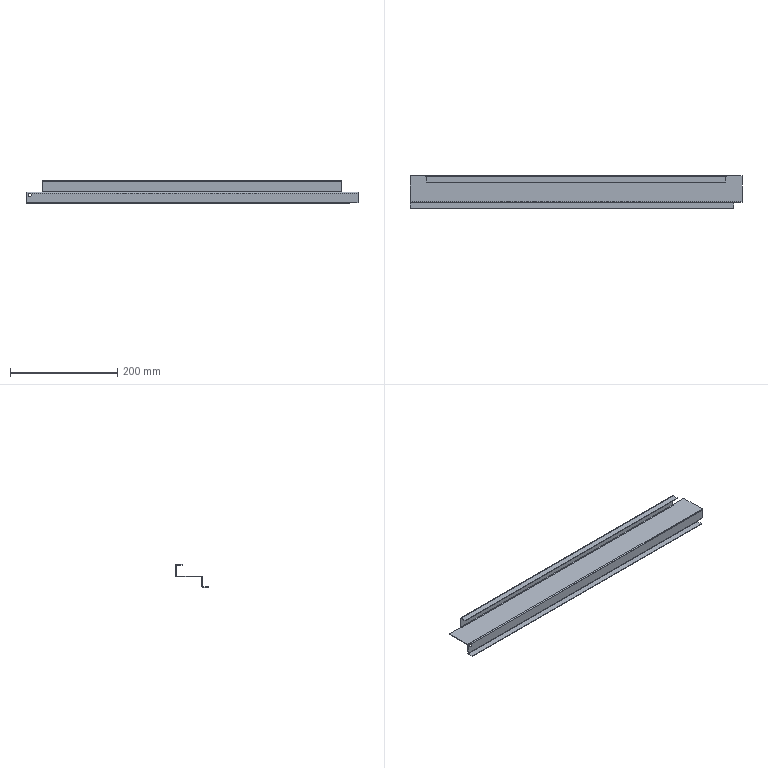Component | SolidWorks | CCQ-1.1-11UpperBeam1-1 | 1 solid | 48 faces | volume 67234 mm3 | plane 38 | cylinder 10 | commonest cylinder face diameters 3.473 x4 1.473 x4 6 x2 | material 304